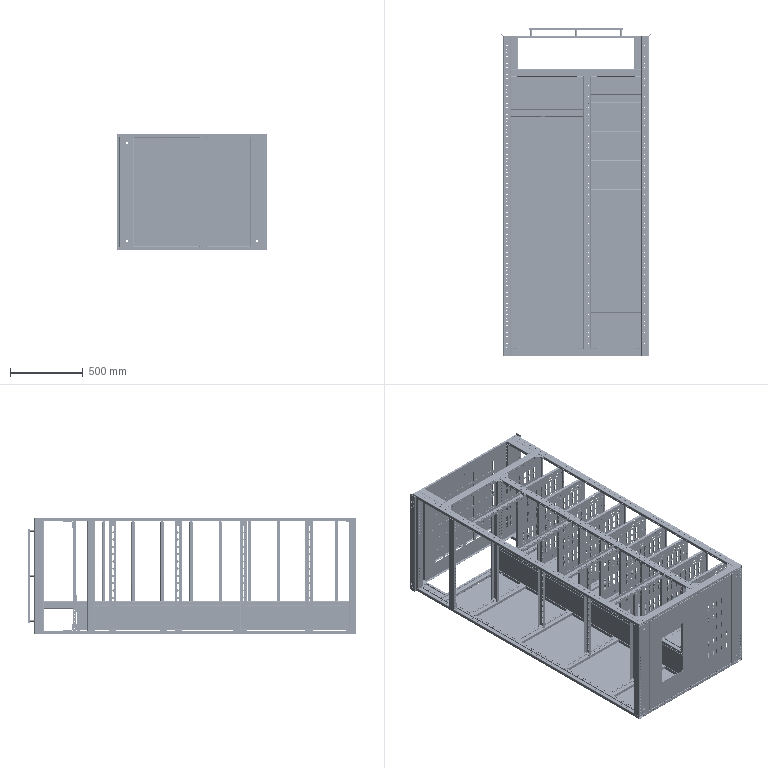Assembly | SolidWorks | mm | 122 component files | 122 solids | 27157 faces | box 1038 x 2260.5 x 800 mm | volume 21110557 mm3 | cylinder 17681 | plane 9064 | spline 208 | torus 204 | commonest cylinder face diameters 5.3 x8368 5 x5113 7.571 x1172 7 x798 9.2 x704 11 x514 2 x317 6 x250
Bill of materials:
BasePlateA | 1 | Plain Carbon Steel | Flat rectangular sheet panel with one large rectangular cutout, an array of narrow vertical slots, and short bent edge returns along two opposite edges. One return is interrupted by a central gap.
CabinetPartitionA | 1 | Plain Carbon Steel | Long, narrow, flat rectangular sheet with continuous upturned flanges along both long edges, forming a shallow open channel/tray.
CabinetPartitionB | 1 | Plain Carbon Steel | Long, flat rectangular sheet with an upturned flange along each long edge. One flange is continuous; the other is split into several separate segments.
CableCompartmentRearPartition | 1 | Plain Carbon Steel | Long sheet-metal channel (C/U section) with a wide web and two short flanges with radiused bends. The flanges have small holes.
C-ChannelPost | 4 | Plain Carbon Steel | Very long, slender lipped channel profile (rectangular section with inward-turned lips leaving a central slot), perforated along its length.
C-ChannelShortPost225 | 4 | Plain Carbon Steel | Short length of lipped channel profile with inward-turned lips forming a slot opening, round holes on the lips and side face, and a notch at one end.
ConnectingPlate | 4 | Plain Carbon Steel | Flat rectangular plate with rounded corners and three round holes. Rounded protrusions appear on the underside at the hole locations.
DoorBeam750 | 1 | Plain Carbon Steel | Tall, vertical lipped channel post with a rounded rectangular section and inward lips. Perforated along its length, with a small notch at one end.
PressurePlate | 16 | Plain Carbon Steel | Solid rectangular/square block plate with five round through-holes in a quincunx pattern (four near the corners and one in the center).
SideBeam900 | 4 | Plain Carbon Steel | Long lipped channel profile (rounded rectangular section with inward lips on one side) with a row of evenly spaced small holes along a side face.
TriangularBracket | 16 | Plain Carbon Steel | Bent sheet corner bracket/gusset: a right-triangular plate with bent flanges along its two perpendicular legs. Each flange has two round holes.
FrontPanel | 2 | Plain Carbon Steel | Long formed sheet profile with a multi-bend section: a horizontal leg, a diagonal segment, a vertical web, and a short return leg. The web has small holes and raised lettering near the ends.
BeamEndPlate | 8 | Plain Carbon Steel | Thin flat rectangular plate with rounded corners and two round through-holes spaced along the long axis.
G-Beam750 | 4 | Plain Carbon Steel | Tall, slender open sheet-metal channel with an asymmetric C-type cross-section. It has two rows of small holes along its length and a larger hole near each end.
HexagonalPost | 8 | Plain Carbon Steel | Hexagonal prism with a round through-bore along its axis. Its shape resembles a hex spacer or standoff.
InsulationSupportBeam | 4 | Plain Carbon Steel | Long, slender sheet-metal post with a closed or nearly closed rectangular section. One face has a single row of evenly spaced elongated slots, and an end face has two round holes.
LayerPartition | 9 | Plain Carbon Steel | Large rectangular sheet-metal panel with return flanges on its edges. It has three bands of vertical elongated slots, each band two rows deep, plus paired short slots, notches and small holes arranged around the field.
MiddleBeam1875 | 3 | Plain Carbon Steel | Very long, slender lipped C-channel with inward-turned lips on the open side. Its faces are densely perforated with small holes along the full length.
MiddleDoorBeam2100 | 1 | Plain Carbon Steel | Very long, slender lipped channel. The open side is on one narrow face, between two short inward lips. A row of small holes runs along one face.
SideBeamA390 | 4 | Plain Carbon Steel | Sheet-metal U-channel or bracket with a flat top web and two side legs. The web runs past the legs at both ends as flat tabs. The web has six obround slots, each flanked by small holes, and each end tab has two holes.
SideBeamB | 8 | Plain Carbon Steel | Sheet-metal U-channel similar to a slotted rail. The web has nine obround slots with pairs of small holes. One end extends as a flat tab with two holes. The other end has a closed end wall or flange with two round holes.
TopCoverA | 1 | Plain Carbon Steel | Thin rectangular plate with a 6 x 6 grid of square cutouts in the centre. Small holes are spread around the perimeter, larger holes sit near the corners, and narrow flanges run along two opposite edges.
TopCoverPlate | 1 | Plain Carbon Steel | Plain, nearly square, thin sheet-metal panel with shallow edge returns. It has eight small holes at the corners and edge midpoints.
TopPartition | 1 | Plain Carbon Steel | Rectangular sheet-metal panel with bent edge flanges. It has three bands of vertical elongated slots, each band two rows deep, and holes in the flanges near the ends.
UpperAndLowerBeam750 | 2 | Plain Carbon Steel | Long, slender, straight profile with a constant cross-section. The section is a rounded rectangle with a central gap in one long side, so it looks like a lipped C-channel or slotted tube. The faces have regularly spaced rows of small round holes along the length, and at least one end has a notch or slot.
WithLocatingConnector | 13 | Plain Carbon Steel | L-shaped bent-plate angle bracket with a 90-degree bend, a rounded inside bend radius and rounded outer corners. One flange has a central round hole with an elongated slot on each side. The other flange has a large central round hole, two plain round holes at opposite corners, and two raised domed bosses or dimples at the other two corners.
Mates:
1. concentric | C-ChannelPost-1 edge at (-5271.503, 8567.064, 6698.842) dir (1, 0, 0) r 2.65 | C-ChannelShortPost225-1 edge at (-5271.503, 8567.064, 6698.842) dir (1, 0, 0) r 2.65
2. coincident | C-ChannelPost-1 face at (-5271.503, 6579.564, 6711.342) dir (1, 0, 0) | C-ChannelShortPost225-1 face at (-5271.503, 8554.564, 6688.342) dir (-1, 0, 0)
3. coincident | C-ChannelPost-2 edge at (-4371.503, 8779.564, 6708.342) dir (0, 0, -1) | C-ChannelShortPost225-2 edge at (-4371.503, 8779.564, 6708.342) dir (0, 0, -1)
4. coincident | C-ChannelPost-2 face at (-4371.503, 8779.564, 6711.342) dir (-1, 0, 0) | C-ChannelShortPost225-2 edge at (-4371.503, 8554.564, 6689.342) dir (0, 0, 1)
5. coincident | C-ChannelPost-2 face at (-4369.503, 6579.564, 6711.342) dir (0, 0, 1) | C-ChannelShortPost225-2 face at (-4373.503, 8554.564, 6711.342) dir (0, 0, 1)
6. coincident | C-ChannelPost-1 face at (-5273.503, 8779.564, 6711.342) dir (0, 0, 1) | SideBeam900-1 face at (-5271.503, 8552.564, 6711.342) dir (0, 0, 1)
7. coincident | C-ChannelShortPost225-1 face at (-5221.503, 8554.564, 6711.342) dir (0, -1, 0) | SideBeam900-1 face at (-5271.503, 8554.564, 6688.342) dir (0, 1, 0)
8. coincident | C-ChannelPost-1 face at (-5271.503, 6579.564, 6711.342) dir (1, 0, 0) | SideBeam900-1 face at (-5271.503, 8504.564, 6711.342) dir (-1, 0, 0)
9. coincident | C-ChannelPost-2 face at (-4371.503, 8779.564, 6711.342) dir (-1, 0, 0) | SideBeam900-1 face at (-4371.503, 8554.564, 6686.342) dir (1, 0, 0)
10. coincident | C-ChannelPost-2 face at (-4369.503, 6579.564, 6711.342) dir (0, 0, 1) | SideBeam900-1 face at (-4371.503, 8506.564, 6711.342) dir (0, 0, 1)
11. coincident | C-ChannelShortPost225-2 edge at (-4421.503, 8554.564, 6708.342) dir (0, 0, -1) | SideBeam900-1 face at (-5271.503, 8554.564, 6688.342) dir (0, 1, 0)
12. coincident | C-ChannelPost-2 face at (-4369.503, 6579.564, 6711.342) dir (0, 0, 1) | SideBeam900-2 face at (-5271.503, 6627.564, 6711.342) dir (0, 0, 1)
13. coincident | C-ChannelPost-2 face at (-4371.503, 8779.564, 6711.342) dir (-1, 0, 0) | SideBeam900-2 face at (-4371.503, 6579.564, 6686.342) dir (1, 0, 0)
14. coincident | C-ChannelPost-2 face at (-4371.503, 6579.564, 6711.342) dir (0, -1, 0) | SideBeam900-2 face at (-4371.503, 6579.564, 6688.342) dir (0, -1, 0)
15. coincident | C-ChannelPost-1 face at (-5273.503, 8779.564, 6711.342) dir (0, 0, 1) | SideBeam900-2 face at (-5271.503, 6627.564, 6711.342) dir (0, 0, 1)
16. coincident | C-ChannelPost-1 face at (-5271.503, 6579.564, 6688.342) dir (0, -1, 0) | SideBeam900-2 face at (-4371.503, 6579.564, 6688.342) dir (0, -1, 0)
17. concentric | C-ChannelShortPost225-1 edge at (-5259.003, 8592.064, 6711.342) dir (0, 0, -1) r 2.65 | ConnectingPlate-1 edge at (-5259.003, 8592.064, 6711.342) dir (0, 0, -1) r 2.65
18. concentric | C-ChannelPost-1 edge at (-5284.003, 8542.064, 6711.342) dir (0, 0, -1) r 2.65 | ConnectingPlate-1 edge at (-5284.003, 8542.064, 6711.342) dir (0, 0, -1) r 2.65
19. coincident | C-ChannelPost-1 face at (-5273.503, 8779.564, 6711.342) dir (0, 0, 1) | ConnectingPlate-1 face at (-5254.503, 8537.564, 6711.342) dir (0, 0, -1)
20. concentric | C-ChannelPost-2 edge at (-4359.003, 8592.064, 6711.342) dir (0, 0, -1) r 2.65 | ConnectingPlate-2 edge at (-4359.003, 8592.064, 6711.342) dir (0, 0, -1) r 2.65
21. concentric | SideBeam900-1 edge at (-4384.003, 8542.064, 6711.342) dir (0, 0, -1) r 2.65 | ConnectingPlate-2 edge at (-4384.003, 8542.064, 6711.342) dir (0, 0, -1) r 2.65
22. coincident | C-ChannelShortPost225-2 face at (-4373.503, 8554.564, 6711.342) dir (0, 0, 1) | ConnectingPlate-2 face at (-4354.503, 8537.564, 6711.342) dir (0, 0, -1)
23. concentric | C-ChannelPost-1 edge at (-5309.003, 8767.064, 6709.342) dir (0, 0, -1) r 2.65 | PressurePlate-1 edge at (-5309.003, 8767.064, 6709.342) dir (0, 0, 1) r 4.5
24. concentric | C-ChannelPost-1 edge at (-5284.003, 8742.064, 6711.342) dir (0, 0, -1) r 2.65 | PressurePlate-1 edge at (-5284.003, 8742.064, 6701.342) dir (0, 0, 1) r 4.5
25. coincident | C-ChannelPost-1 face at (-5273.503, 8779.564, 6709.342) dir (0, 0, -1) | PressurePlate-1 face at (-5319.003, 8734.564, 6709.342) dir (0, 0, 1)
26. concentric | C-ChannelShortPost225-1 edge at (-5259.003, 8767.064, 6711.342) dir (0, 0, -1) r 2.65 | PressurePlate-2 edge at (-5259.003, 8767.064, 6709.342) dir (0, 0, 1) r 4.5
27. concentric | C-ChannelShortPost225-1 edge at (-5234.003, 8742.064, 6711.342) dir (0, 0, -1) r 2.65 | PressurePlate-2 edge at (-5234.003, 8742.064, 6709.342) dir (0, 0, 1) r 4.5
28. coincident | C-ChannelShortPost225-1 face at (-5223.503, 8779.564, 6709.342) dir (0, 0, -1) | PressurePlate-2 face at (-5269.003, 8734.564, 6709.342) dir (0, 0, 1)
29. concentric | C-ChannelShortPost225-2 edge at (-4409.003, 8767.064, 6711.342) dir (0, 0, -1) r 2.65 | PressurePlate-3 edge at (-4409.003, 8767.064, 6709.342) dir (0, 0, 1) r 4.5
30. concentric | C-ChannelShortPost225-2 edge at (-4384.003, 8742.064, 6711.342) dir (0, 0, -1) r 2.65 | PressurePlate-3 edge at (-4384.003, 8742.064, 6709.342) dir (0, 0, 1) r 4.5
31. coincident | C-ChannelShortPost225-2 face at (-4373.503, 8554.564, 6709.342) dir (0, 0, -1) | PressurePlate-3 face at (-4419.003, 8734.564, 6709.342) dir (0, 0, 1)
32. concentric | C-ChannelPost-2 edge at (-4359.003, 8767.064, 6711.342) dir (0, 0, -1) r 2.65 | PressurePlate-4 edge at (-4359.003, 8767.064, 6709.342) dir (0, 0, 1) r 4.5
33. concentric | C-ChannelPost-2 edge at (-4334.003, 8742.064, 6711.342) dir (0, 0, -1) r 2.65 | PressurePlate-4 edge at (-4334.003, 8742.064, 6709.342) dir (0, 0, 1) r 4.5
34. coincident | C-ChannelPost-2 face at (-4323.503, 8779.564, 6709.342) dir (0, 0, -1) | PressurePlate-4 face at (-4369.003, 8734.564, 6709.342) dir (0, 0, 1)
35. concentric | C-ChannelPost-1 edge at (-5271.503, 8467.064, 6698.842) dir (1, 0, 0) r 2.65 | TriangularBracket-1 edge at (-5271.503, 8467.064, 6698.842) dir (-1, 0, 0) r 3.5
36. concentric | SideBeam900-1 edge at (-5234.003, 8504.564, 6698.842) dir (0, 1, 0) r 2.65 | TriangularBracket-1 edge at (-5234.003, 8504.564, 6698.842) dir (0, 1, 0) r 3.5
37. concentric | C-ChannelPost-2 edge at (-4371.503, 8467.064, 6698.842) dir (-1, 0, 0) r 2.65 | TriangularBracket-2 edge at (-4371.503, 8467.064, 6698.842) dir (1, 0, 0) r 3.5
38. concentric | SideBeam900-1 edge at (-4409.003, 8504.564, 6698.842) dir (0, 1, 0) r 2.65 | TriangularBracket-2 edge at (-4409.003, 8502.564, 6698.842) dir (0, 1, 0) r 3.5
39. concentric | C-ChannelPost-1 edge at (-5271.503, 6667.064, 6698.842) dir (1, 0, 0) r 2.65 | TriangularBracket-3 edge at (-5271.503, 6667.064, 6698.842) dir (-1, 0, 0) r 3.5
40. concentric | SideBeam900-2 edge at (-5234.003, 6629.564, 6698.842) dir (0, -1, 0) r 2.65 | TriangularBracket-3 edge at (-5234.003, 6631.564, 6698.842) dir (0, -1, 0) r 3.5
41. concentric | C-ChannelPost-2 edge at (-4371.503, 6667.064, 6698.842) dir (-1, 0, 0) r 2.65 | TriangularBracket-4 edge at (-4371.503, 6667.064, 6698.842) dir (1, 0, 0) r 3.5
42. concentric | SideBeam900-2 edge at (-4409.003, 6629.564, 6698.842) dir (0, -1, 0) r 2.65 | TriangularBracket-4 edge at (-4409.003, 6629.564, 6698.842) dir (0, -1, 0) r 3.5
43. concentric | C-ChannelPost-1 edge at (-5309.003, 6617.064, 6711.342) dir (0, 0, -1) r 2.65 | PressurePlate-5 edge at (-5309.003, 6617.064, 6709.342) dir (0, 0, 1) r 4.5
44. concentric | C-ChannelPost-1 edge at (-5284.003, 6592.064, 6711.342) dir (0, 0, -1) r 2.65 | PressurePlate-5 edge at (-5284.003, 6592.064, 6709.342) dir (0, 0, 1) r 4.5
45. coincident | C-ChannelPost-1 face at (-5273.503, 8779.564, 6709.342) dir (0, 0, -1) | PressurePlate-5 face at (-5319.003, 6584.564, 6709.342) dir (0, 0, 1)
46. concentric | SideBeam900-2 edge at (-5259.003, 6617.064, 6711.342) dir (0, 0, -1) r 2.65 | PressurePlate-6 edge at (-5259.003, 6617.064, 6709.342) dir (0, 0, 1) r 4.5
47. concentric | SideBeam900-2 edge at (-5234.003, 6592.064, 6711.342) dir (0, 0, -1) r 2.65 | PressurePlate-6 edge at (-5234.003, 6592.064, 6709.342) dir (0, 0, 1) r 4.5
48. coincident | SideBeam900-2 face at (-4371.503, 6581.564, 6709.342) dir (0, 0, -1) | PressurePlate-6 face at (-5269.003, 6584.564, 6709.342) dir (0, 0, 1)
49. concentric | C-ChannelPost-2 edge at (-4334.003, 6617.064, 6711.342) dir (0, 0, -1) r 2.65 | PressurePlate-7 edge at (-4334.003, 6617.064, 6709.342) dir (0, 0, 1) r 4.5
50. concentric | C-ChannelPost-2 edge at (-4359.003, 6592.064, 6711.342) dir (0, 0, -1) r 2.65 | PressurePlate-7 edge at (-4359.003, 6592.064, 6709.342) dir (0, 0, 1) r 4.5
51. coincident | C-ChannelPost-2 face at (-4323.503, 8779.564, 6709.342) dir (0, 0, -1) | PressurePlate-7 face at (-4369.003, 6584.564, 6709.342) dir (0, 0, 1)
52. concentric | SideBeam900-2 edge at (-4384.003, 6617.064, 6711.342) dir (0, 0, -1) r 2.65 | PressurePlate-8 edge at (-4384.003, 6617.064, 6709.342) dir (0, 0, 1) r 4.5
53. concentric | SideBeam900-2 edge at (-4409.003, 6592.064, 6711.342) dir (0, 0, -1) r 2.65 | PressurePlate-8 edge at (-4409.003, 6592.064, 6709.342) dir (0, 0, 1) r 4.5
54. coincident | SideBeam900-2 face at (-5271.503, 6627.564, 6709.342) dir (0, 0, -1) | PressurePlate-8 face at (-4419.003, 6584.564, 6709.342) dir (0, 0, 1)
55. concentric | PressurePlate-4 edge at (-4346.503, 8754.564, 6709.342) dir (0, 0, 1) r 4.25 | G-Beam-1/BeamEndPlate-1 edge at (-4346.503, 8754.564, 6711.342) dir (0, 0, -1) r 5.5
56. concentric | PressurePlate-3 edge at (-4396.503, 8754.564, 6709.342) dir (0, 0, 1) r 4.25 | G-Beam-1/BeamEndPlate-1 edge at (-4396.503, 8754.564, 6711.342) dir (0, 0, -1) r 5.5
57. coincident | C-ChannelPost-2 face at (-4323.503, 8779.564, 6711.342) dir (0, 0, 1) | G-Beam-1/G-Beam750-1 face at (-4321.503, 8776.564, 6711.342) dir (0, 0, -1)
58. concentric | PressurePlate-7 edge at (-4346.503, 6604.564, 6709.342) dir (0, 0, 1) r 4.25 | G-Beam-2/BeamEndPlate-2 edge at (-4346.503, 6604.564, 6716.342) dir (0, 0, -1) r 5.5
59. concentric | PressurePlate-8 edge at (-4396.503, 6604.564, 6709.342) dir (0, 0, 1) r 4.25 | G-Beam-2/BeamEndPlate-2 edge at (-4396.503, 6604.564, 6716.342) dir (0, 0, -1) r 5.5
60. coincident | C-ChannelPost-2 face at (-4369.503, 6579.564, 6711.342) dir (0, 0, 1) | G-Beam-2/G-Beam750-1 face at (-4324.503, 6629.564, 6711.342) dir (0, 0, -1)
61. concentric | PressurePlate-1 edge at (-5296.503, 8754.564, 6709.342) dir (0, 0, 1) r 4.25 | G-Beam-3/BeamEndPlate-2 edge at (-5296.503, 8754.564, 6711.342) dir (0, 0, -1) r 5.5
62. concentric | PressurePlate-2 edge at (-5246.503, 8754.564, 6709.342) dir (0, 0, 1) r 4.25 | G-Beam-3/BeamEndPlate-2 edge at (-5246.503, 8754.564, 6711.342) dir (0, 0, -1) r 5.5
63. coincident | C-ChannelPost-1 face at (-5319.503, 6579.564, 6711.342) dir (0, 0, 1) | G-Beam-3/G-Beam750-1 face at (-5321.503, 8776.564, 6711.342) dir (0, 0, -1)
64. concentric | PressurePlate-6 edge at (-5246.503, 6604.564, 6709.342) dir (0, 0, 1) r 4.25 | G-Beam-4/BeamEndPlate-1 edge at (-5246.503, 6604.564, 6716.342) dir (0, 0, -1) r 5.5
65. concentric | PressurePlate-5 edge at (-5296.503, 6604.564, 6709.342) dir (0, 0, 1) r 4.25 | G-Beam-4/BeamEndPlate-1 edge at (-5296.503, 6604.564, 6711.342) dir (0, 0, -1) r 5.5
66. coincident | C-ChannelPost-1 face at (-5319.503, 6579.564, 6711.342) dir (0, 0, 1) | G-Beam-4/G-Beam750-1 face at (-5276.503, 6629.564, 6711.342) dir (0, 0, -1)
67. concentric | G-Beam-3/BeamEndPlate-1 edge at (-5296.503, 8754.564, 7461.342) dir (0, 0, 1) r 5.5 | Frame-1/PressurePlate-4 edge at (-5296.503, 8754.564, 7463.342) dir (0, 0, -1) r 4.25
68. concentric | G-Beam-3/BeamEndPlate-1 edge at (-5246.503, 8754.564, 7461.342) dir (0, 0, 1) r 5.5 | Frame-1/PressurePlate-3 edge at (-5246.503, 8754.564, 7463.342) dir (0, 0, -1) r 4.25
69. concentric | G-Beam-1/BeamEndPlate-2 edge at (-4396.503, 8754.564, 7461.342) dir (0, 0, 1) r 5.5 | Frame-1/PressurePlate-2 edge at (-4396.503, 8754.564, 7463.342) dir (0, 0, -1) r 4.25
70. concentric | G-Beam-1/BeamEndPlate-2 edge at (-4346.503, 8754.564, 7461.342) dir (0, 0, 1) r 5.5 | Frame-1/PressurePlate-1 edge at (-4346.503, 8754.564, 7463.342) dir (0, 0, -1) r 4.25
71. coincident | G-Beam-4/G-Beam750-1 face at (-5318.503, 6629.564, 7461.342) dir (0, 0, 1) | Frame-1/C-ChannelPost-2 face at (-5319.503, 8779.564, 7461.342) dir (0, 0, -1)
72. concentric | Frame-1/TriangularBracket-3 edge at (-4373.503, 6642.064, 7473.842) dir (1, 0, 0) r 3.5 | MiddleBeam1875-2 edge at (-4721.503, 6642.064, 7473.842) dir (-1, 0, 0) r 2.65
73. distance | Frame-1/C-ChannelPost-1 face at (-4321.503, 8779.564, 7461.342) dir (1, 0, 0) | MiddleBeam1875-2 face at (-4723.503, 6629.564, 7484.342) dir (-1, 0, 0)
74. concentric | TriangularBracket-2 edge at (-4373.503, 8492.064, 6698.842) dir (1, 0, 0) r 3.5 | MiddleBeam1875-3 edge at (-4721.503, 8492.064, 6698.842) dir (-1, 0, 0) r 2.65
75. concentric | MiddleBeam1875-2 edge at (-4734.003, 8492.064, 7461.342) dir (0, 0, 1) r 2.65 | MiddleBeam1875-3 edge at (-4734.003, 8492.064, 6686.342) dir (0, 0, -1) r 3.785
76. concentric | MiddleBeam1875-2 edge at (-4734.003, 6642.064, 7461.342) dir (0, 0, 1) r 2.65 | MiddleBeam1875-3 edge at (-4734.003, 6642.064, 6686.342) dir (0, 0, -1) r 3.785
77. concentric | Frame-1/SideBeam900-1 edge at (-4684.003, 8504.564, 7473.842) dir (0, 1, 0) r 2.65 | TriangularBracket-5 edge at (-4684.003, 8502.564, 7473.842) dir (0, 1, 0) r 3.5
78. concentric | Frame-1/SideBeam900-2 edge at (-4684.003, 6629.564, 7473.842) dir (0, -1, 0) r 2.65 | TriangularBracket-6 edge at (-4684.003, 6631.564, 7473.842) dir (0, -1, 0) r 3.5
79. concentric | Frame-1/SideBeam900-2 edge at (-4809.003, 6629.564, 7473.842) dir (0, -1, 0) r 2.65 | TriangularBracket-8 edge at (-4809.003, 6631.564, 7473.842) dir (0, -1, 0) r 3.5
80. concentric | Frame-1/SideBeam900-1 edge at (-4809.003, 8504.564, 7473.842) dir (0, 1, 0) r 2.65 | assembly edge at (584.851, 1094.637, -254.55) dir (0.4049, -0.7384, 0.5393) r 3.5
81. concentric | MiddleBeam1875-2 edge at (590.956, 1145.912, -254.758) dir (0.5461, 0.6684, 0.505) r 2.65 | assembly edge at (589.863, 1144.576, -255.768) dir (0.5461, 0.6684, 0.505) r 3.5
82. concentric | Frame-1/SideBeam900-1 edge at (-4809.003, 8504.564, 7473.842) dir (0, 1, 0) r 2.65 | TriangularBracket-9 edge at (-4809.003, 8504.564, 7473.842) dir (0, 1, 0) r 3.5
83. concentric | SideBeam900-1 edge at (-4809.003, 8504.564, 6698.842) dir (0, 1, 0) r 2.65 | TriangularBracket-10 edge at (-4809.003, 8502.564, 6698.842) dir (0, 1, 0) r 3.5
84. concentric | MiddleBeam1875-3 edge at (-4721.503, 8492.064, 6698.842) dir (-1, 0, 0) r 2.65 | TriangularBracket-11 edge at (-4719.503, 8492.064, 6698.842) dir (-1, 0, 0) r 3.5
85. concentric | SideBeam900-1 edge at (-4684.003, 8504.564, 6698.842) dir (0, 1, 0) r 2.65 | TriangularBracket-11 edge at (-4684.003, 8502.564, 6698.842) dir (0, 1, 0) r 3.5
86. concentric | SideBeam900-2 edge at (-4684.003, 6629.564, 6698.842) dir (0, -1, 0) r 2.65 | TriangularBracket-12 edge at (-4684.003, 6631.564, 6698.842) dir (0, -1, 0) r 3.5
87. concentric | SideBeam900-2 edge at (-4809.003, 6629.564, 6698.842) dir (0, -1, 0) r 2.65 | TriangularBracket-13 edge at (-4809.003, 6631.564, 6698.842) dir (0, -1, 0) r 3.5
88. coincident | G-Beam-1/G-Beam750-1 face at (-4321.503, 8729.564, 6711.342) dir (1, 0, 0) | FrontPanel-1 face at (-4321.503, 8748.52, 7486.342) dir (-1, 0, 0)
89. coincident | G-Beam-1/G-Beam750-1 face at (-4421.503, 8779.564, 6711.342) dir (0, 1, 0) | FrontPanel-1 face at (-4321.458, 8779.564, 7486.342) dir (0, -1, 0)
90. coincident | C-ChannelPost-2 face at (-4321.503, 8779.564, 6686.342) dir (0, 0, -1) | FrontPanel-1 face at (-4304.503, 8748.52, 6686.342) dir (0, 0, -1)
91. coincident | Frame-1/SideBeam900-2 face at (-5271.503, 6629.564, 7484.342) dir (0, 1, 0) | UpperAndLowerBeam750-2 face at (-4721.503, 6629.564, 6711.342) dir (0, 1, 0)
92. distance | SideBeam900-2 face at (-4371.503, 6581.564, 6711.342) dir (0, 0, 1) | UpperAndLowerBeam750-2 face at (-4721.503, 6604.564, 6711.342) dir (0, 0, -1)
93. distance | G-Beam-2/G-Beam750-1 face at (-4321.503, 6629.564, 7461.342) dir (1, 0, 0) | UpperAndLowerBeam750-2 face at (-4721.503, 6627.564, 7461.342) dir (1, 0, 0)
94. distance | Frame-1/SideBeam900-1 face at (-4371.503, 8504.564, 7484.342) dir (0, -1, 0) | UpperAndLowerBeam750-3 face at (-4771.503, 8504.564, 6711.342) dir (0, -1, 0)
95. distance | SideBeam900-1 face at (-4371.503, 8506.564, 6711.342) dir (0, 0, 1) | UpperAndLowerBeam750-3 face at (-4721.503, 8506.564, 6711.342) dir (0, 0, -1)
96. distance | Frame-1/C-ChannelPost-1 face at (-4321.503, 8779.564, 7461.342) dir (1, 0, 0) | UpperAndLowerBeam750-3 face at (-4721.503, 8506.564, 6711.342) dir (1, 0, 0)
97. concentric | TriangularBracket-5 edge at (-4719.503, 8467.064, 7473.842) dir (-1, 0, 0) r 3.5 | MiddleBeam1875-2 edge at (-4721.503, 8467.064, 7473.842) dir (-1, 0, 0) r 2.65
98. concentric | TriangularBracket-6 edge at (-4719.503, 6667.064, 7473.842) dir (-1, 0, 0) r 3.5 | MiddleBeam1875-2 edge at (-4723.503, 6667.064, 7473.842) dir (-1, 0, 0) r 2.65
99. concentric | TriangularBracket-8 edge at (-4773.503, 6667.064, 7473.842) dir (1, 0, 0) r 3.5 | MiddleBeam1875-2 edge at (-4771.503, 6667.064, 7473.842) dir (1, 0, 0) r 2.65
100. concentric | MiddleBeam1875-3 edge at (-4721.503, 6667.064, 6698.842) dir (-1, 0, 0) r 2.65 | TriangularBracket-12 edge at (-4719.503, 6667.064, 6698.842) dir (-1, 0, 0) r 3.5
101. concentric | MiddleBeam1875-3 edge at (-4769.503, 6667.064, 6698.842) dir (1, 0, 0) r 2.65 | TriangularBracket-13 edge at (-4773.503, 6667.064, 6698.842) dir (1, 0, 0) r 3.5
102. concentric | MiddleBeam1875-2 edge at (-4771.503, 8492.064, 7473.842) dir (1, 0, 0) r 2.65 | TriangularBracket-9 edge at (-4773.503, 8492.064, 7473.842) dir (1, 0, 0) r 3.5
103. concentric | MiddleBeam1875-3 edge at (-4771.503, 8467.064, 6698.842) dir (1, 0, 0) r 2.65 | TriangularBracket-10 edge at (-4773.503, 8467.064, 6698.842) dir (1, 0, 0) r 3.5
104. concentric | MiddleBeam1875-2 edge at (-4734.003, 8492.064, 7461.342) dir (0, 0, 1) r 2.65 | MiddleBeam1875-4 edge at (-4734.003, 8492.064, 6886.342) dir (0, 0, -1) r 3.785
105. concentric | MiddleBeam1875-2 edge at (-4759.003, 6642.064, 7461.342) dir (0, 0, 1) r 2.65 | MiddleBeam1875-4 edge at (-4759.003, 6642.064, 6886.342) dir (0, 0, -1) r 3.785
106. distance | MiddleBeam1875-2 face at (-4771.503, 6629.564, 7486.342) dir (0, 0, 1) | MiddleBeam1875-4 face at (-4723.503, 8504.564, 6911.342) dir (0, 0, 1)
107. coincident | Frame-1/SideBeam900-2 face at (-5271.503, 6629.564, 7484.342) dir (0, 1, 0) | MiddleBeam1875-2 edge at (-4723.503, 6629.564, 7464.342) dir (0, 0, 1)
108. coincident | Frame-1/SideBeam900-1 face at (-4371.503, 8504.564, 7484.342) dir (0, -1, 0) | MiddleBeam1875-2 edge at (-4769.503, 8504.564, 7464.342) dir (0, 0, 1)
109. coincident | SideBeam900-2 face at (-4371.503, 6629.564, 6688.342) dir (0, 1, 0) | MiddleBeam1875-3 edge at (-4769.503, 6629.564, 6708.342) dir (0, 0, -1)
110. coincident | SideBeam900-1 face at (-5271.503, 8504.564, 6688.342) dir (0, -1, 0) | MiddleBeam1875-3 edge at (-4723.503, 8504.564, 6708.342) dir (0, 0, -1)
111. concentric | UpperAndLowerBeam750-3 edge at (-4734.003, 8529.564, 7423.842) dir (0, -1, 0) r 2.65 | WithLocatingConnector-1 edge at (-4734.003, 8532.564, 7423.842) dir (0, 1, 0) r 3.5
112. concentric | UpperAndLowerBeam750-3 edge at (-4759.003, 8529.564, 7448.842) dir (0, -1, 0) r 2.65 | WithLocatingConnector-1 edge at (-4759.003, 8532.564, 7448.842) dir (0, 1, 0) r 3.5
113. coincident | UpperAndLowerBeam750-3 face at (-4723.503, 8529.564, 6711.342) dir (0, 1, 0) | WithLocatingConnector-1 face at (-4766.003, 8529.564, 7417.342) dir (0, -1, 0)
114. concentric | UpperAndLowerBeam750-3 edge at (-4759.003, 8529.564, 6748.842) dir (0, -1, 0) r 2.65 | WithLocatingConnector-2 edge at (-4759.003, 8532.564, 6748.842) dir (0, 1, 0) r 3.5
115. concentric | UpperAndLowerBeam750-3 edge at (-4734.003, 8529.564, 6723.842) dir (0, -1, 0) r 2.65 | WithLocatingConnector-2 edge at (-4734.003, 8529.564, 6723.842) dir (0, 1, 0) r 3.5
116. coincident | UpperAndLowerBeam750-3 face at (-4769.503, 8529.564, 6711.342) dir (0, 1, 0) | WithLocatingConnector-2 face at (-4727.003, 8529.564, 6755.342) dir (0, -1, 0)
117. concentric | UpperAndLowerBeam750-2 edge at (-4734.003, 6629.564, 7423.842) dir (0, 1, 0) r 3.785 | WithLocatingConnector-3 edge at (-4734.003, 6632.564, 7423.842) dir (0, 1, 0) r 3.5
118. concentric | UpperAndLowerBeam750-2 edge at (-4759.003, 6629.564, 7448.842) dir (0, 1, 0) r 3.785 | WithLocatingConnector-3 edge at (-4759.003, 6632.564, 7448.842) dir (0, 1, 0) r 3.5
119. coincident | UpperAndLowerBeam750-2 face at (-4721.503, 6629.564, 6711.342) dir (0, 1, 0) | WithLocatingConnector-3 face at (-4766.003, 6629.564, 7417.342) dir (0, -1, 0)
120. concentric | UpperAndLowerBeam750-2 edge at (-4734.003, 6629.564, 6848.842) dir (0, 1, 0) r 3.785 | WithLocatingConnector-4 edge at (-4734.003, 6632.564, 6848.842) dir (0, 1, 0) r 3.5
121. concentric | UpperAndLowerBeam750-2 edge at (-4759.003, 6629.564, 6873.842) dir (0, 1, 0) r 3.785 | WithLocatingConnector-4 edge at (-4759.003, 6632.564, 6873.842) dir (0, 1, 0) r 3.5
122. coincident | UpperAndLowerBeam750-2 face at (-4721.503, 6629.564, 6711.342) dir (0, 1, 0) | WithLocatingConnector-4 face at (-4766.003, 6629.564, 6842.342) dir (0, -1, 0)
123. concentric | UpperAndLowerBeam750-2 edge at (-4759.003, 6629.564, 6748.842) dir (0, 1, 0) r 3.785 | WithLocatingConnector-5 edge at (-4759.003, 6632.564, 6748.842) dir (0, 1, 0) r 3.5
124. concentric | UpperAndLowerBeam750-2 edge at (-4734.003, 6629.564, 6723.842) dir (0, 1, 0) r 3.785 | WithLocatingConnector-5 edge at (-4734.003, 6632.564, 6723.842) dir (0, 1, 0) r 3.5
125. coincident | UpperAndLowerBeam750-2 face at (-4721.503, 6629.564, 6711.342) dir (0, 1, 0) | WithLocatingConnector-5 face at (-4727.003, 6629.564, 6755.342) dir (0, -1, 0)
126. concentric | UpperAndLowerBeam750-3 edge at (-4734.003, 8504.564, 6748.842) dir (0, -1, 0) r 3.785 | WithLocatingConnector-6 edge at (-4734.003, 8504.564, 6748.842) dir (0, -1, 0) r 3.5
127. concentric | UpperAndLowerBeam750-3 edge at (-4759.003, 8504.564, 6723.842) dir (0, -1, 0) r 3.785 | WithLocatingConnector-6 edge at (-4759.003, 8501.564, 6723.842) dir (0, -1, 0) r 3.5
128. coincident | UpperAndLowerBeam750-3 face at (-4771.503, 8504.564, 6711.342) dir (0, -1, 0) | WithLocatingConnector-6 face at (-4766.003, 8504.564, 6755.342) dir (0, 1, 0)
129. concentric | UpperAndLowerBeam750-3 edge at (-4759.003, 8504.564, 6848.842) dir (0, -1, 0) r 3.785 | WithLocatingConnector-7 edge at (-4759.003, 8501.564, 6848.842) dir (0, -1, 0) r 3.5
130. concentric | UpperAndLowerBeam750-3 edge at (-4734.003, 8504.564, 6873.842) dir (0, -1, 0) r 3.785 | WithLocatingConnector-7 edge at (-4734.003, 8501.564, 6873.842) dir (0, -1, 0) r 3.5
131. coincident | UpperAndLowerBeam750-3 face at (-4771.503, 8504.564, 6711.342) dir (0, -1, 0) | WithLocatingConnector-7 face at (-4727.003, 8504.564, 6842.342) dir (0, 1, 0)
132. concentric | UpperAndLowerBeam750-3 edge at (-4734.003, 8504.564, 6948.842) dir (0, -1, 0) r 3.785 | WithLocatingConnector-8 edge at (-4734.003, 8501.564, 6948.842) dir (0, -1, 0) r 3.5
133. concentric | UpperAndLowerBeam750-3 edge at (-4759.003, 8504.564, 6923.842) dir (0, -1, 0) r 3.785 | WithLocatingConnector-8 edge at (-4759.003, 8501.564, 6923.842) dir (0, -1, 0) r 3.5
134. coincident | UpperAndLowerBeam750-3 face at (-4771.503, 8504.564, 6711.342) dir (0, -1, 0) | WithLocatingConnector-8 face at (-4766.003, 8504.564, 6955.342) dir (0, 1, 0)
135. concentric | UpperAndLowerBeam750-2 edge at (-4759.003, 6629.564, 6948.842) dir (0, 1, 0) r 3.785 | WithLocatingConnector-9 edge at (-4759.003, 6632.564, 6948.842) dir (0, 1, 0) r 3.5
136. concentric | UpperAndLowerBeam750-2 edge at (-4734.003, 6629.564, 6923.842) dir (0, 1, 0) r 3.785 | WithLocatingConnector-9 edge at (-4734.003, 6632.564, 6923.842) dir (0, 1, 0) r 3.5
137. coincident | UpperAndLowerBeam750-2 face at (-4721.503, 6629.564, 6711.342) dir (0, 1, 0) | WithLocatingConnector-9 face at (-4727.003, 6629.564, 6955.342) dir (0, -1, 0)
138. concentric | Frame-1/C-ChannelPost-1 edge at (-4334.003, 6642.064, 7461.342) dir (0, 0, 1) r 2.65 | MiddleDoorBeam2100-1 edge at (-4334.003, 6642.064, 6911.342) dir (0, 0, -1) r 2.65
139. concentric | Frame-1/C-ChannelPost-1 edge at (-4334.003, 8717.064, 7461.342) dir (0, 0, 1) r 2.65 | MiddleDoorBeam2100-1 edge at (-4334.003, 8717.064, 6911.342) dir (0, 0, -1) r 2.65
140. distance | Frame-1/C-ChannelPost-1 face at (-4321.503, 6579.564, 7486.342) dir (0, 0, 1) | MiddleDoorBeam2100-1 face at (-4323.503, 8729.564, 6911.342) dir (0, 0, 1)
141. concentric | MiddleDoorBeam2100-1 edge at (-4346.503, 8692.064, 6873.842) dir (1, 0, 0) r 2.65 | WithLocatingConnector-10 edge at (-4349.503, 8692.064, 6873.842) dir (-1, 0, 0) r 3.5
142. concentric | MiddleDoorBeam2100-1 edge at (-4346.503, 8717.064, 6898.842) dir (1, 0, 0) r 2.65 | WithLocatingConnector-10 edge at (-4349.503, 8717.064, 6898.842) dir (-1, 0, 0) r 3.5
143. coincident | MiddleDoorBeam2100-1 face at (-4346.503, 6629.564, 6909.342) dir (-1, 0, 0) | WithLocatingConnector-10 face at (-4346.503, 8685.564, 6905.842) dir (1, 0, 0)
144. concentric | MiddleDoorBeam2100-1 edge at (-4346.503, 6667.064, 6898.842) dir (1, 0, 0) r 2.65 | WithLocatingConnector-11 edge at (-4346.503, 6667.064, 6898.842) dir (-1, 0, 0) r 3.5
145. concentric | MiddleDoorBeam2100-1 edge at (-4346.503, 6642.064, 6873.842) dir (1, 0, 0) r 2.65 | WithLocatingConnector-11 edge at (-4346.503, 6642.064, 6873.842) dir (-1, 0, 0) r 3.5
146. concentric | MiddleDoorBeam2100-1 edge at (-4346.503, 6667.064, 6898.842) dir (1, 0, 0) r 2.65 | WithLocatingConnector-11 edge at (-4346.503, 6667.064, 6898.842) dir (-1, 0, 0) r 3.5
147. concentric | MiddleDoorBeam2100-1 edge at (-4346.503, 6642.064, 6873.842) dir (1, 0, 0) r 2.65 | WithLocatingConnector-11 edge at (-4349.503, 6642.064, 6873.842) dir (-1, 0, 0) r 3.5
148. coincident | MiddleDoorBeam2100-1 face at (-4346.503, 6629.564, 6909.342) dir (-1, 0, 0) | WithLocatingConnector-11 face at (-4346.503, 6673.564, 6866.842) dir (1, 0, 0)
149. concentric | G-Beam-3/G-Beam750-1 edge at (-5271.503, 8779.564, 6748.842) dir (0, -1, 0) r 9 | TopCoverA-2 edge at (-5271.503, 8781.564, 6748.842) dir (0, -1, 0) r 9
150. concentric | G-Beam-1/G-Beam750-1 edge at (-4371.503, 8779.564, 7423.842) dir (0, -1, 0) r 9 | TopCoverA-2 edge at (-4371.503, 8781.564, 7423.842) dir (0, -1, 0) r 9
151. coincident | G-Beam-1/G-Beam750-1 face at (-4421.503, 8779.564, 6711.342) dir (0, 1, 0) | TopCoverA-2 face at (-5221.503, 8779.564, 6688.842) dir (0, -1, 0)
152. concentric | G-Beam-3/G-Beam750-1 edge at (-5309.003, 8779.564, 6723.842) dir (0, -1, 0) r 2.65 | FrontPanel-2 edge at (-5309.003, 8781.564, 6723.842) dir (0, 1, 0) r 3.5
153. concentric | G-Beam-3/G-Beam750-1 edge at (-5309.003, 8779.564, 7448.842) dir (0, -1, 0) r 2.65 | FrontPanel-2 edge at (-5309.003, 8781.564, 7448.842) dir (0, 1, 0) r 3.5
154. coincident | G-Beam-3/G-Beam750-1 face at (-5221.503, 8779.564, 7461.342) dir (0, 1, 0) | FrontPanel-2 face at (-5321.548, 8779.564, 6686.342) dir (0, -1, 0)
155. concentric | SideBeam900-2 edge at (-5159.003, 6592.064, 6711.342) dir (0, 0, -1) r 2.65 | BasePlateA-1 edge at (-5159.003, 6592.064, 6713.842) dir (0, 0, -1) r 3.5
156. concentric | Frame-1/SideBeam900-2 edge at (-5159.003, 6592.064, 7461.342) dir (0, 0, 1) r 2.65 | BasePlateA-1 edge at (-5159.003, 6592.064, 7460.842) dir (0, 0, 1) r 3.5
157. concentric | SideBeam900-2 edge at (-4484.003, 6592.064, 6711.342) dir (0, 0, -1) r 2.65 | BasePlateA-1 edge at (-4484.003, 6592.064, 6713.842) dir (0, 0, -1) r 3.5
158. concentric | Frame-1/SideBeam900-2 edge at (-4484.003, 6592.064, 7461.342) dir (0, 0, 1) r 2.65 | BasePlateA-1 edge at (-4484.003, 6592.064, 7460.842) dir (0, 0, 1) r 3.5
159. distance | Frame-1/SideBeam900-2 face at (-5271.503, 6581.564, 7461.342) dir (0, 0, -1) | BasePlateA-1 face at (-4697.003, 6599.564, 7460.842) dir (0, 0, 1)
160. concentric | TopCoverA-2 edge at (-4511.757, 8781.564, 7396.342) dir (0, -1, 0) r 3.5 | HexagonalPost-1 edge at (-4511.757, 8781.564, 7396.342) dir (0, 1, 0) r 3.5
161. concentric | HexagonalPost-1 edge at (-4511.757, 8838.564, 7396.342) dir (0, 1, 0) r 3.5 | TopCoverPlate-1 edge at (-4511.757, 8840.064, 7396.342) dir (0, -1, 0) r 3.5
162. concentric | HexagonalPost-9 edge at (-5131.757, 8838.564, 6776.342) dir (0, 1, 0) r 3.5 | TopCoverPlate-1 edge at (-5131.757, 8840.064, 6776.342) dir (0, -1, 0) r 3.5
163. coincident | HexagonalPost-9 face at (-5136.986, 8838.564, 6773.896) dir (0, 1, 0) | TopCoverPlate-1 face at (-5146.757, 8838.564, 6761.342) dir (0, -1, 0)
164. coincident | MiddleDoorBeam2100-1 face at (-4323.503, 8729.564, 6911.342) dir (0, 0, 1) | LayerPartition-12 face at (-4768.503, 6725.064, 6911.342) dir (0, 0, -1)
165. concentric | MiddleBeam1875-2 edge at (-4759.003, 6717.064, 7461.342) dir (0, 0, 1) r 2.65 | LayerPartition-12 edge at (-4759.003, 6717.064, 7459.342) dir (0, 0, -1) r 3.5
166. concentric | MiddleBeam1875-4 edge at (-4759.003, 6717.064, 6911.342) dir (0, 0, -1) r 2.65 | LayerPartition-12 edge at (-4759.003, 6717.064, 6913.342) dir (0, 0, -1) r 3.5
167. concentric | UpperAndLowerBeam750-3 edge at (-4721.503, 8518.064, 6923.842) dir (-1, 0, 0) r 2.65 | TopPartition-10 edge at (-4721.503, 8518.064, 6923.842) dir (1, 0, 0) r 3.5
168. concentric | UpperAndLowerBeam750-3 edge at (-4721.503, 8518.064, 7448.842) dir (-1, 0, 0) r 2.65 | TopPartition-10 edge at (-4721.503, 8518.064, 7448.842) dir (1, 0, 0) r 3.5
169. coincident | Frame-1/C-ChannelPost-1 face at (-4321.503, 8779.564, 7461.342) dir (1, 0, 0) | TopPartition-10 face at (-4321.503, 8528.564, 6914.342) dir (1, 0, 0)
170. concentric | C-ChannelPost-2 edge at (-4359.003, 6892.064, 6711.342) dir (0, 0, -1) r 2.65 | SideBeamA390-1 edge at (-4359.003, 6892.064, 6713.842) dir (0, 0, -1) r 3.5
171. concentric | C-ChannelPost-2 edge at (-4359.003, 6917.064, 6711.342) dir (0, 0, -1) r 2.65 | SideBeamA390-1 edge at (-4359.003, 6917.064, 6713.842) dir (0, 0, -1) r 3.5
172. coincident | MiddleBeam1875-3 face at (-4723.503, 8504.564, 6711.342) dir (0, 0, 1) | SideBeamA390-1 face at (-4376.503, 6879.564, 6711.342) dir (0, 0, -1)
173. concentric | MiddleBeam1875-3 edge at (-4771.503, 6917.064, 6698.842) dir (1, 0, 0) r 2.65 | SideBeamB-1 edge at (-4774.003, 6917.064, 6698.842) dir (1, 0, 0) r 3.5
174. concentric | MiddleBeam1875-3 edge at (-4771.503, 6892.064, 6698.842) dir (1, 0, 0) r 2.65 | SideBeamB-1 edge at (-4774.003, 6892.064, 6698.842) dir (1, 0, 0) r 3.5
175. concentric | C-ChannelPost-1 edge at (-5284.003, 6892.064, 6711.342) dir (0, 0, -1) r 2.65 | SideBeamB-1 edge at (-5284.003, 6892.064, 6711.342) dir (0, 0, -1) r 3.5
176. concentric | MiddleBeam1875-2 edge at (-4771.503, 6917.064, 7473.842) dir (1, 0, 0) r 2.65 | SideBeamB-5 edge at (-4774.003, 6917.064, 7473.842) dir (1, 0, 0) r 3.5
177. concentric | Frame-1/C-ChannelPost-1 edge at (-4371.503, 6892.064, 7473.842) dir (-1, 0, 0) r 2.65 | SideBeamB-5 edge at (-4774.003, 6892.064, 7473.842) dir (1, 0, 0) r 3.5
178. concentric | Frame-1/C-ChannelPost-2 edge at (-5284.003, 6892.064, 7461.342) dir (0, 0, 1) r 2.65 | SideBeamB-5 edge at (-5284.003, 6892.064, 7458.842) dir (0, 0, 1) r 3.5
179. coincident | SideBeamB-5 face at (-5266.503, 6879.564, 7458.842) dir (0, 0, -1) | InsulationSupportBeam-1 face at (-5059.003, 6883.064, 7458.842) dir (0, 0, 1)
180. concentric | SideBeamB-1 edge at (-5046.503, 6917.064, 6713.842) dir (0, 0, -1) r 2.65 | InsulationSupportBeam-1 edge at (-5046.503, 6917.064, 6717.342) dir (0, 0, -1) r 3.5
181. concentric | SideBeamB-5 edge at (-5046.503, 6917.064, 7458.842) dir (0, 0, 1) r 2.65 | InsulationSupportBeam-1 edge at (-5046.503, 6917.064, 7456.342) dir (0, 0, 1) r 3.5
182. concentric | G-Beam-3/G-Beam750-1 edge at (-5309.003, 8729.564, 6723.842) dir (0, 1, 0) r 2.65 | DoorBeam750-1 edge at (-5309.003, 8429.564, 6723.842) dir (0, -1, 0) r 2.65
183. concentric | G-Beam-3/G-Beam750-1 edge at (-5309.003, 8729.564, 7448.842) dir (0, 1, 0) r 2.65 | DoorBeam750-1 edge at (-5309.003, 8429.564, 7448.842) dir (0, -1, 0) r 2.65
184. distance | G-Beam-3/G-Beam750-1 face at (-5318.503, 8729.564, 6711.342) dir (0, -1, 0) | DoorBeam750-1 face at (-5320.503, 8429.564, 7461.342) dir (0, 1, 0)
185. concentric | DoorBeam750-1 edge at (-5297.503, 8417.064, 7448.842) dir (-1, 0, 0) r 2.65 | WithLocatingConnector-12 edge at (-5294.503, 8417.064, 7448.842) dir (1, 0, 0) r 3.5
186. concentric | DoorBeam750-1 edge at (-5297.503, 8392.064, 7423.842) dir (-1, 0, 0) r 2.65 | WithLocatingConnector-12 edge at (-5294.503, 8392.064, 7423.842) dir (1, 0, 0) r 3.5
187. coincident | DoorBeam750-1 face at (-5297.503, 8427.564, 7461.342) dir (1, 0, 0) | WithLocatingConnector-12 face at (-5297.503, 8424.064, 7417.342) dir (-1, 0, 0)
188. concentric | DoorBeam750-1 edge at (-5297.503, 8417.064, 6748.842) dir (-1, 0, 0) r 2.65 | WithLocatingConnector-13 edge at (-5294.503, 8417.064, 6748.842) dir (1, 0, 0) r 3.5
189. concentric | DoorBeam750-1 edge at (-5297.503, 8392.064, 6723.842) dir (-1, 0, 0) r 2.65 | WithLocatingConnector-13 edge at (-5294.503, 8392.064, 6723.842) dir (1, 0, 0) r 3.5
190. coincident | DoorBeam750-1 face at (-5297.503, 8427.564, 7461.342) dir (1, 0, 0) | WithLocatingConnector-13 face at (-5297.503, 8385.064, 6755.342) dir (-1, 0, 0)
191. concentric | C-ChannelPost-2 edge at (-4371.503, 8392.064, 6698.842) dir (-1, 0, 0) r 2.65 | CabinetPartitionA-1 edge at (-4372.003, 8392.064, 6698.842) dir (1, 0, 0) r 3.5
192. concentric | C-ChannelPost-2 edge at (-4371.503, 6742.064, 6698.842) dir (-1, 0, 0) r 2.65 | CabinetPartitionA-1 edge at (-4372.003, 6742.064, 6698.842) dir (1, 0, 0) r 3.5
193. distance | C-ChannelPost-2 face at (-4371.503, 8779.564, 6711.342) dir (-1, 0, 0) | CabinetPartitionA-1 face at (-4372.003, 6678.064, 6710.842) dir (1, 0, 0)
194. concentric | MiddleBeam1875-3 edge at (-4771.503, 6742.064, 6698.842) dir (1, 0, 0) r 2.65 | CabinetPartitionB-1 edge at (-4772.003, 6742.064, 6698.842) dir (-1, 0, 0) r 3.5
195. concentric | C-ChannelPost-1 edge at (-5271.503, 8392.064, 6698.842) dir (1, 0, 0) r 2.65 | CabinetPartitionB-1 edge at (-5271.003, 8392.064, 6698.842) dir (1, 0, 0) r 3.5
196. distance | MiddleBeam1875-3 face at (-4771.503, 6629.564, 6688.342) dir (-1, 0, 0) | CabinetPartitionB-1 face at (-4772.003, 8456.064, 6710.842) dir (1, 0, 0)
197. concentric | MiddleBeam1875-3 edge at (-4759.003, 6742.064, 6711.342) dir (0, 0, -1) r 2.65 | CableCompartmentRearPartition-1 edge at (-4759.003, 6742.064, 6711.842) dir (0, 0, -1) r 3.5
198. concentric | MiddleBeam1875-3 edge at (-4759.003, 8392.064, 6711.342) dir (0, 0, -1) r 2.65 | CableCompartmentRearPartition-1 edge at (-4759.003, 8392.064, 6713.342) dir (0, 0, -1) r 3.5
199. distance | MiddleBeam1875-4 face at (-4721.503, 6629.564, 6886.342) dir (0, 0, -1) | CableCompartmentRearPartition-1 face at (-4751.503, 8479.064, 6885.842) dir (0, 0, 1)
200. concentric | C-ChannelPost-1 edge at (1416.784, 1380.989, -275.785) dir (-0.5389, -0.777, -0.3253) r 2.65 | C-ChannelShortPost225-1 edge at (1416.784, 1380.989, -275.785) dir (-0.5389, -0.777, -0.3253) r 2.65
201. coincident | C-ChannelPost-1 face at (-218.712, 2510.292, -263.965) dir (-0.5389, -0.777, -0.3253) | C-ChannelShortPost225-1 face at (1408.459, 1390.92, -285.714) dir (0.5389, 0.777, 0.3253)
202. coincident | C-ChannelPost-2 edge at (1104.645, 558.028, -559.6) dir (0.1854, 0.2673, -0.9456) | C-ChannelShortPost225-2 edge at (1104.645, 558.028, -559.6) dir (0.1854, 0.2673, -0.9456)
203. coincident | C-ChannelPost-2 face at (1104.089, 557.226, -556.763) dir (0.5389, 0.777, 0.3253) | C-ChannelShortPost225-2 edge at (923.28, 691.331, -577.567) dir (-0.1854, -0.2673, 0.9456)
204. coincident | C-ChannelPost-2 face at (-704.784, 1809.418, -557.414) dir (-0.1854, -0.2673, 0.9456) | C-ChannelShortPost225-2 face at (920.279, 687.004, -556.113) dir (-0.1854, -0.2673, 0.9456)
205. coincident | C-ChannelPost-1 face at (1590.161, 1258.101, -263.314) dir (-0.1854, -0.2673, 0.9456) | SideBeam900-1 face at (1402.552, 1385.911, -263.965) dir (-0.1854, -0.2673, 0.9456)
206. coincident | C-ChannelShortPost225-1 face at (1377.251, 1345.92, -280.232) dir (-0.8217, 0.5699, 0) | SideBeam900-1 face at (1408.459, 1390.92, -285.714) dir (0.8217, -0.5699, 0)
207. coincident | C-ChannelPost-1 face at (-218.712, 2510.292, -263.965) dir (-0.5389, -0.777, -0.3253) | SideBeam900-1 face at (1363.109, 1413.265, -263.965) dir (0.5389, 0.777, 0.3253)
208. coincident | C-ChannelPost-2 face at (1104.089, 557.226, -556.763) dir (0.5389, 0.777, 0.3253) | SideBeam900-1 face at (923.836, 692.133, -580.403) dir (-0.5389, -0.777, -0.3253)
209. coincident | C-ChannelPost-2 face at (-704.784, 1809.418, -557.414) dir (-0.1854, -0.2673, 0.9456) | SideBeam900-1 face at (879.758, 712.805, -556.763) dir (-0.1854, -0.2673, 0.9456)
210. coincident | C-ChannelShortPost225-2 edge at (946.701, 725.103, -543.334) dir (0.1854, 0.2673, -0.9456) | SideBeam900-1 face at (1408.459, 1390.92, -285.714) dir (0.8217, -0.5699, 0)
211. coincident | C-ChannelPost-2 face at (-704.784, 1809.418, -557.414) dir (-0.1854, -0.2673, 0.9456) | SideBeam900-2 face at (-179.269, 2482.938, -263.965) dir (-0.1854, -0.2673, 0.9456)
212. coincident | C-ChannelPost-2 face at (1104.089, 557.226, -556.763) dir (0.5389, 0.777, 0.3253) | SideBeam900-2 face at (-699.071, 1817.655, -580.403) dir (-0.5389, -0.777, -0.3253)
213. coincident | C-ChannelPost-2 face at (-703.706, 1810.972, -556.763) dir (-0.8217, 0.5699, 0) | SideBeam900-2 face at (-699.442, 1817.12, -578.512) dir (-0.8217, 0.5699, 0)
214. coincident | C-ChannelPost-1 face at (1590.161, 1258.101, -263.314) dir (-0.1854, -0.2673, 0.9456) | SideBeam900-2 face at (-179.269, 2482.938, -263.965) dir (-0.1854, -0.2673, 0.9456)
215. coincident | C-ChannelPost-1 face at (-214.447, 2516.441, -285.714) dir (-0.8217, 0.5699, 0) | SideBeam900-2 face at (-699.442, 1817.12, -578.512) dir (-0.8217, 0.5699, 0)
216. concentric | C-ChannelShortPost225-1 edge at (1428.274, 1353.688, -268.032) dir (0.1854, 0.2673, -0.9456) r 2.65 | ConnectingPlate-1 edge at (1428.274, 1353.688, -268.032) dir (0.1854, 0.2673, -0.9456) r 2.65
217. concentric | C-ChannelPost-1 edge at (1400.66, 1401.607, -259.898) dir (0.1854, 0.2673, -0.9456) r 2.65 | ConnectingPlate-1 edge at (1400.66, 1401.607, -259.898) dir (0.1854, 0.2673, -0.9456) r 2.65
218. coincident | C-ChannelPost-1 face at (1590.161, 1258.101, -263.314) dir (-0.1854, -0.2673, 0.9456) | ConnectingPlate-1 face at (1381.065, 1381.25, -269.496) dir (0.1854, 0.2673, -0.9456)
219. concentric | C-ChannelPost-2 edge at (943.28, 654.367, -560.83) dir (0.1854, 0.2673, -0.9456) r 2.65 | ConnectingPlate-2 edge at (943.28, 654.367, -560.83) dir (0.1854, 0.2673, -0.9456) r 2.65
220. concentric | SideBeam900-1 edge at (915.665, 702.286, -552.697) dir (0.1854, 0.2673, -0.9456) r 2.65 | ConnectingPlate-2 edge at (915.665, 702.286, -552.697) dir (0.1854, 0.2673, -0.9456) r 2.65
221. coincident | C-ChannelShortPost225-2 face at (920.279, 687.004, -556.113) dir (-0.1854, -0.2673, 0.9456) | ConnectingPlate-2 face at (896.071, 681.929, -562.294) dir (0.1854, 0.2673, -0.9456)
222. concentric | C-ChannelPost-1 edge at (1599.391, 1293.344, -253.656) dir (0.1854, 0.2673, -0.9456) r 2.65 | PressurePlate-1 edge at (1599.391, 1293.344, -253.656) dir (-0.1854, -0.2673, 0.9456) r 4.5
223. concentric | C-ChannelPost-1 edge at (1565.005, 1287.63, -259.898) dir (0.1854, 0.2673, -0.9456) r 2.65 | PressurePlate-1 edge at (1566.859, 1290.304, -269.354) dir (-0.1854, -0.2673, 0.9456) r 4.5
224. coincident | C-ChannelPost-1 face at (1590.532, 1258.636, -265.206) dir (0.1854, 0.2673, -0.9456) | PressurePlate-1 face at (1578.073, 1319.635, -250.403) dir (-0.1854, -0.2673, 0.9456)
225. concentric | C-ChannelShortPost225-1 edge at (1572.076, 1253.958, -268.032) dir (0.1854, 0.2673, -0.9456) r 2.65 | PressurePlate-2 edge at (1572.447, 1254.492, -269.923) dir (-0.1854, -0.2673, 0.9456) r 4.5
226. concentric | C-ChannelShortPost225-1 edge at (1538.061, 1248.779, -276.165) dir (0.1854, 0.2673, -0.9456) r 2.65 | PressurePlate-2 edge at (1538.431, 1249.314, -278.056) dir (-0.1854, -0.2673, 0.9456) r 4.5
227. coincident | C-ChannelShortPost225-1 face at (1563.588, 1219.785, -281.472) dir (0.1854, 0.2673, -0.9456) | PressurePlate-2 face at (1551.129, 1280.784, -266.67) dir (-0.1854, -0.2673, 0.9456)
228. concentric | C-ChannelShortPost225-2 edge at (1114.026, 593.488, -544.564) dir (0.1854, 0.2673, -0.9456) r 2.65 | PressurePlate-3 edge at (1114.396, 594.023, -546.455) dir (-0.1854, -0.2673, 0.9456) r 4.5
229. concentric | C-ChannelShortPost225-2 edge at (1080.01, 588.31, -552.697) dir (0.1854, 0.2673, -0.9456) r 2.65 | PressurePlate-3 edge at (1080.381, 588.844, -554.588) dir (-0.1854, -0.2673, 0.9456) r 4.5
230. coincident | C-ChannelShortPost225-2 face at (920.649, 687.539, -558.004) dir (0.1854, 0.2673, -0.9456) | PressurePlate-3 face at (1093.079, 620.314, -543.201) dir (-0.1854, -0.2673, 0.9456)
231. concentric | C-ChannelPost-2 edge at (1087.081, 554.637, -560.83) dir (0.1854, 0.2673, -0.9456) r 2.65 | PressurePlate-4 edge at (1087.452, 555.172, -562.721) dir (-0.1854, -0.2673, 0.9456) r 4.5
232. concentric | C-ChannelPost-2 edge at (1053.066, 549.458, -568.963) dir (0.1854, 0.2673, -0.9456) r 2.65 | PressurePlate-4 edge at (1053.437, 549.993, -570.855) dir (-0.1854, -0.2673, 0.9456) r 4.5
233. coincident | C-ChannelPost-2 face at (1078.593, 520.464, -574.271) dir (0.1854, 0.2673, -0.9456) | PressurePlate-4 face at (1066.135, 581.463, -559.468) dir (-0.1854, -0.2673, 0.9456)
234. concentric | C-ChannelPost-1 edge at (1334.612, 1437.978, -275.785) dir (-0.5389, -0.777, -0.3253) r 2.65 | TriangularBracket-1 edge at (1334.612, 1437.978, -275.785) dir (0.5389, 0.777, 0.3253) r 3.5
235. concentric | SideBeam900-1 edge at (1345.218, 1387.468, -287.985) dir (0.8217, -0.5699, 0) r 2.65 | TriangularBracket-1 edge at (1345.218, 1387.468, -287.985) dir (0.8217, -0.5699, 0) r 3.5
236. concentric | C-ChannelPost-2 edge at (849.617, 738.657, -568.583) dir (0.5389, 0.777, 0.3253) r 2.65 | TriangularBracket-2 edge at (849.617, 738.657, -568.583) dir (-0.5389, -0.777, -0.3253) r 3.5
237. concentric | SideBeam900-1 edge at (900.64, 746.424, -556.384) dir (0.8217, -0.5699, 0) r 2.65 | TriangularBracket-2 edge at (898.997, 747.564, -556.384) dir (0.8217, -0.5699, 0) r 3.5
238. concentric | C-ChannelPost-1 edge at (-144.493, 2463.769, -275.785) dir (-0.5389, -0.777, -0.3253) r 2.65 | TriangularBracket-3 edge at (-144.493, 2463.769, -275.785) dir (0.5389, 0.777, 0.3253) r 3.5
239. concentric | SideBeam900-2 edge at (-195.516, 2456.001, -287.985) dir (-0.8217, 0.5699, 0) r 2.65 | TriangularBracket-3 edge at (-193.873, 2454.862, -287.985) dir (-0.8217, 0.5699, 0) r 3.5
240. concentric | C-ChannelPost-2 edge at (-629.488, 1764.448, -568.583) dir (0.5389, 0.777, 0.3253) r 2.65 | TriangularBracket-4 edge at (-629.488, 1764.448, -568.583) dir (-0.5389, -0.777, -0.3253) r 3.5
241. concentric | SideBeam900-2 edge at (-640.094, 1814.957, -556.384) dir (-0.8217, 0.5699, 0) r 2.65 | TriangularBracket-4 edge at (-640.094, 1814.957, -556.384) dir (-0.8217, 0.5699, 0) r 3.5
242. concentric | C-ChannelPost-1 edge at (-167.689, 2518.06, -251.765) dir (0.1854, 0.2673, -0.9456) r 2.65 | PressurePlate-5 edge at (-167.318, 2518.595, -253.656) dir (-0.1854, -0.2673, 0.9456) r 4.5
243. concentric | C-ChannelPost-1 edge at (-201.704, 2512.882, -259.898) dir (0.1854, 0.2673, -0.9456) r 2.65 | PressurePlate-5 edge at (-201.333, 2513.416, -261.79) dir (-0.1854, -0.2673, 0.9456) r 4.5
244. coincident | C-ChannelPost-1 face at (1590.532, 1258.636, -265.206) dir (0.1854, 0.2673, -0.9456) | PressurePlate-5 face at (-188.635, 2544.886, -250.403) dir (-0.1854, -0.2673, 0.9456)
245. concentric | SideBeam900-2 edge at (-194.633, 2479.209, -268.032) dir (0.1854, 0.2673, -0.9456) r 2.65 | PressurePlate-6 edge at (-194.262, 2479.744, -269.923) dir (-0.1854, -0.2673, 0.9456) r 4.5
246. concentric | SideBeam900-2 edge at (-228.648, 2474.03, -276.165) dir (0.1854, 0.2673, -0.9456) r 2.65 | PressurePlate-6 edge at (-228.277, 2474.565, -278.056) dir (-0.1854, -0.2673, 0.9456) r 4.5
247. coincident | SideBeam900-2 face at (-701.692, 1810.366, -558.655) dir (0.1854, 0.2673, -0.9456) | PressurePlate-6 face at (-215.579, 2506.035, -266.67) dir (-0.1854, -0.2673, 0.9456)
248. concentric | C-ChannelPost-2 edge at (-693.099, 1760.463, -568.963) dir (0.1854, 0.2673, -0.9456) r 2.65 | PressurePlate-7 edge at (-692.729, 1760.997, -570.855) dir (-0.1854, -0.2673, 0.9456) r 4.5
249. concentric | C-ChannelPost-2 edge at (-700.17, 1794.135, -560.83) dir (0.1854, 0.2673, -0.9456) r 2.65 | PressurePlate-7 edge at (-699.8, 1794.67, -562.721) dir (-0.1854, -0.2673, 0.9456) r 4.5
250. coincident | C-ChannelPost-2 face at (1078.593, 520.464, -574.271) dir (0.1854, 0.2673, -0.9456) | PressurePlate-7 face at (-700.574, 1806.714, -559.468) dir (-0.1854, -0.2673, 0.9456)
251. concentric | SideBeam900-2 edge at (-666.155, 1799.314, -552.697) dir (0.1854, 0.2673, -0.9456) r 2.65 | PressurePlate-8 edge at (-665.784, 1799.848, -554.588) dir (-0.1854, -0.2673, 0.9456) r 4.5
252. concentric | SideBeam900-2 edge at (-673.226, 1832.986, -544.564) dir (0.1854, 0.2673, -0.9456) r 2.65 | PressurePlate-8 edge at (-672.856, 1833.521, -546.455) dir (-0.1854, -0.2673, 0.9456) r 4.5
253. coincident | SideBeam900-2 face at (-178.898, 2483.473, -265.856) dir (0.1854, 0.2673, -0.9456) | PressurePlate-8 face at (-673.63, 1845.565, -543.201) dir (-0.1854, -0.2673, 0.9456)
254. concentric | C-ChannelPost-1 edge at (1582.207, 1268.566, -275.134) dir (-0.5389, -0.777, -0.3253) r 2.65 | C-ChannelShortPost225-1 edge at (1580.051, 1265.458, -276.436) dir (-0.5389, -0.777, -0.3253) r 2.65
255. coincident | G-Beam750-1 face at (-301.487, -43.193, -36.523) dir (0, 0, 1) | BeamEndPlate-1 face at (-301.487, -134.193, -36.523) dir (0, 0, -1)
256. distance | G-Beam750-1 face at (-301.487, -140.193, 10.477) dir (0, 1, 0) | BeamEndPlate-1 face at (-301.487, -139.193, -31.523) dir (0, -1, 0)
257. coincident | G-Beam750-1 face at (-301.487, -43.193, -19.523) dir (-1, 0, 0) | BeamEndPlate-1 face at (-301.487, -52.193, 2.477) dir (-1, 0, 0)
258. coincident | G-Beam750-1 face at (448.513, -140.193, 10.477) dir (1, 0, 0) | BeamEndPlate-2 face at (448.513, -52.193, -31.523) dir (1, 0, 0)
259. distance | G-Beam750-1 face at (448.513, -46.193, -19.523) dir (0, -1, 0) | BeamEndPlate-2 face at (448.513, -47.193, 2.477) dir (0, 1, 0)
260. coincident | G-Beam750-1 face at (-301.487, -43.193, -36.523) dir (0, 0, 1) | BeamEndPlate-2 face at (448.513, -134.193, -36.523) dir (0, 0, -1)